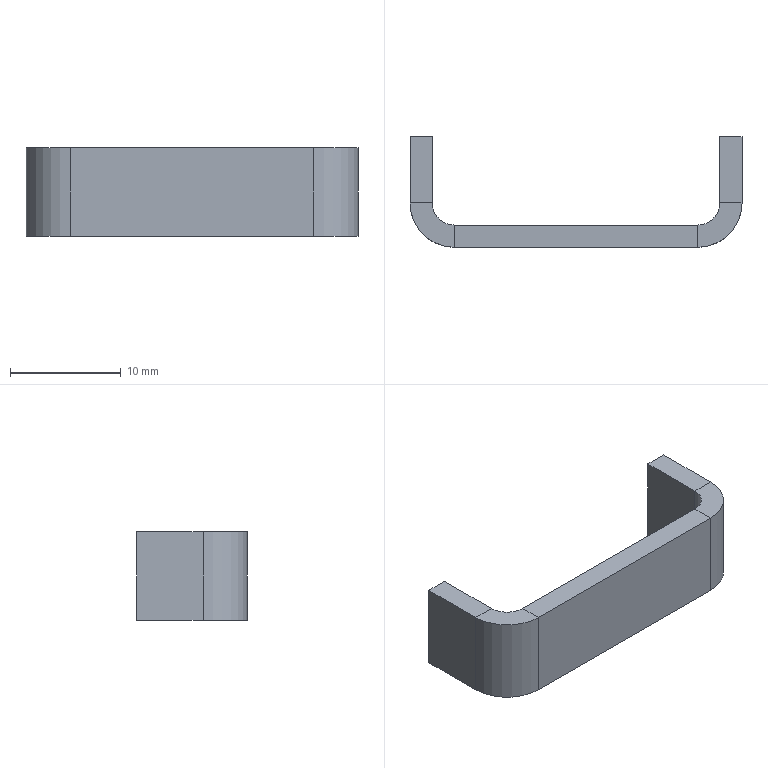Component | SolidWorks | ElectricalCabinetAssembly-1_ControlPanelAssembly-1_CableClamp-1 | 1 solid | 22 faces | box 30 x 10 x 8 mm | volume 695 mm3 | plane 18 | cylinder 4 | commonest cylinder face diameters 8 x2 4 x2 | material Plain Carbon Steel
STEP:
#1=COLOUR_RGB('',0.7922,0.8196,0.9333);
#2=FILL_AREA_STYLE_COLOUR('',#1);
#3=FILL_AREA_STYLE('',(#2));
#4=SURFACE_STYLE_FILL_AREA(#3);
#5=SURFACE_SIDE_STYLE('',(#4));
#6=SURFACE_STYLE_USAGE(.BOTH.,#5);
#7=PRESENTATION_STYLE_ASSIGNMENT((#6));
#8=CARTESIAN_POINT('',(86.921,47.384,67.696));
#9=VERTEX_POINT('',#8);
#10=CARTESIAN_POINT('',(86.921,47.463,67.696));
#11=VERTEX_POINT('',#10);
#12=CARTESIAN_POINT('',(86.921,47.384,67.696));
#13=DIRECTION('',(-0.,1.,0.));
#14=VECTOR('',#13,39.37);
#15=LINE('',#12,#14);
#16=EDGE_CURVE('',#9,#11,#15,.T.);
#17=ORIENTED_EDGE('',*,*,#16,.F.);
#18=CARTESIAN_POINT('',(86.763,47.541,67.696));
#19=VERTEX_POINT('',#18);
#20=CARTESIAN_POINT('',(86.921,47.541,67.696));
#21=DIRECTION('',(0.,-0.,1.));
#22=DIRECTION('',(1.,0.,0.));
#23=AXIS2_PLACEMENT_3D('',#20,#21,#22);
#24=CIRCLE('',#23,0.1575);
#25=EDGE_CURVE('',#19,#9,#24,.T.);
#26=ORIENTED_EDGE('',*,*,#25,.F.);
#27=CARTESIAN_POINT('',(86.842,47.541,67.696));
#28=VERTEX_POINT('',#27);
#29=CARTESIAN_POINT('',(86.842,47.541,67.696));
#30=DIRECTION('',(-1.,-0.,0.));
#31=VECTOR('',#30,39.37);
#32=LINE('',#29,#31);
#33=EDGE_CURVE('',#28,#19,#32,.T.);
#34=ORIENTED_EDGE('',*,*,#33,.F.);
#35=CARTESIAN_POINT('',(86.921,47.541,67.696));
#36=DIRECTION('',(0.,-0.,1.));
#37=DIRECTION('',(1.,0.,0.));
#38=AXIS2_PLACEMENT_3D('',#35,#36,#37);
#39=CIRCLE('',#38,0.07874);
#40=EDGE_CURVE('',#28,#11,#39,.T.);
#41=ORIENTED_EDGE('',*,*,#40,.T.);
#42=EDGE_LOOP('',(#17,#26,#34,#41));
#43=FACE_OUTER_BOUND('',#42,.T.);
#44=CARTESIAN_POINT('',(86.921,47.384,67.696));
#45=DIRECTION('',(-0.,0.,-1.));
#46=DIRECTION('',(1.,0.,-0.));
#47=AXIS2_PLACEMENT_3D('',#44,#45,#46);
#48=PLANE('',#47);
#49=ADVANCED_FACE('',(#43),#48,.T.);
#50=CARTESIAN_POINT('',(87.787,47.384,67.696));
#51=VERTEX_POINT('',#50);
#52=CARTESIAN_POINT('',(86.763,47.384,67.696));
#53=DIRECTION('',(1.,0.,-0.));
#54=VECTOR('',#53,39.37);
#55=LINE('',#52,#54);
#56=EDGE_CURVE('',#9,#51,#55,.T.);
#57=ORIENTED_EDGE('',*,*,#56,.F.);
#58=ORIENTED_EDGE('',*,*,#16,.T.);
#59=CARTESIAN_POINT('',(87.787,47.463,67.696));
#60=VERTEX_POINT('',#59);
#61=CARTESIAN_POINT('',(86.763,47.463,67.696));
#62=DIRECTION('',(1.,0.,-0.));
#63=VECTOR('',#62,39.37);
#64=LINE('',#61,#63);
#65=EDGE_CURVE('',#11,#60,#64,.T.);
#66=ORIENTED_EDGE('',*,*,#65,.T.);
#67=CARTESIAN_POINT('',(87.787,47.463,67.696));
#68=DIRECTION('',(0.,-1.,-0.));
#69=VECTOR('',#68,39.37);
#70=LINE('',#67,#69);
#71=EDGE_CURVE('',#60,#51,#70,.T.);
#72=ORIENTED_EDGE('',*,*,#71,.T.);
#73=EDGE_LOOP('',(#57,#58,#66,#72));
#74=FACE_OUTER_BOUND('',#73,.T.);
#75=CARTESIAN_POINT('',(86.842,47.541,67.696));
#76=DIRECTION('',(-0.,0.,-1.));
#77=DIRECTION('',(1.,0.,-0.));
#78=AXIS2_PLACEMENT_3D('',#75,#76,#77);
#79=PLANE('',#78);
#80=ADVANCED_FACE('',(#74),#79,.T.);
#81=CARTESIAN_POINT('',(86.763,47.541,68.011));
#82=VERTEX_POINT('',#81);
#83=CARTESIAN_POINT('',(86.842,47.541,68.011));
#84=VERTEX_POINT('',#83);
#85=CARTESIAN_POINT('',(86.763,47.541,68.011));
#86=DIRECTION('',(1.,0.,-0.));
#87=VECTOR('',#86,39.37);
#88=LINE('',#85,#87);
#89=EDGE_CURVE('',#82,#84,#88,.T.);
#90=ORIENTED_EDGE('',*,*,#89,.F.);
#91=CARTESIAN_POINT('',(86.921,47.384,68.011));
#92=VERTEX_POINT('',#91);
#93=CARTESIAN_POINT('',(86.921,47.541,68.011));
#94=DIRECTION('',(0.,-0.,1.));
#95=DIRECTION('',(1.,0.,0.));
#96=AXIS2_PLACEMENT_3D('',#93,#94,#95);
#97=CIRCLE('',#96,0.1575);
#98=EDGE_CURVE('',#82,#92,#97,.T.);
#99=ORIENTED_EDGE('',*,*,#98,.T.);
#100=CARTESIAN_POINT('',(86.921,47.463,68.011));
#101=VERTEX_POINT('',#100);
#102=CARTESIAN_POINT('',(86.921,47.463,68.011));
#103=DIRECTION('',(0.,-1.,-0.));
#104=VECTOR('',#103,39.37);
#105=LINE('',#102,#104);
#106=EDGE_CURVE('',#101,#92,#105,.T.);
#107=ORIENTED_EDGE('',*,*,#106,.F.);
#108=CARTESIAN_POINT('',(86.921,47.541,68.011));
#109=DIRECTION('',(0.,-0.,1.));
#110=DIRECTION('',(1.,0.,0.));
#111=AXIS2_PLACEMENT_3D('',#108,#109,#110);
#112=CIRCLE('',#111,0.07874);
#113=EDGE_CURVE('',#84,#101,#112,.T.);
#114=ORIENTED_EDGE('',*,*,#113,.F.);
#115=EDGE_LOOP('',(#90,#99,#107,#114));
#116=FACE_OUTER_BOUND('',#115,.T.);
#117=CARTESIAN_POINT('',(86.763,47.541,68.011));
#118=DIRECTION('',(0.,-0.,1.));
#119=DIRECTION('',(-1.,-0.,0.));
#120=AXIS2_PLACEMENT_3D('',#117,#118,#119);
#121=PLANE('',#120);
#122=ADVANCED_FACE('',(#116),#121,.T.);
#123=CARTESIAN_POINT('',(86.763,47.778,68.011));
#124=VERTEX_POINT('',#123);
#125=CARTESIAN_POINT('',(86.763,47.778,68.011));
#126=DIRECTION('',(0.,-1.,-0.));
#127=VECTOR('',#126,39.37);
#128=LINE('',#125,#127);
#129=EDGE_CURVE('',#124,#82,#128,.T.);
#130=ORIENTED_EDGE('',*,*,#129,.T.);
#131=ORIENTED_EDGE('',*,*,#89,.T.);
#132=CARTESIAN_POINT('',(86.842,47.778,68.011));
#133=VERTEX_POINT('',#132);
#134=CARTESIAN_POINT('',(86.842,47.778,68.011));
#135=DIRECTION('',(0.,-1.,-0.));
#136=VECTOR('',#135,39.37);
#137=LINE('',#134,#136);
#138=EDGE_CURVE('',#133,#84,#137,.T.);
#139=ORIENTED_EDGE('',*,*,#138,.F.);
#140=CARTESIAN_POINT('',(86.842,47.778,68.011));
#141=DIRECTION('',(-1.,-0.,0.));
#142=VECTOR('',#141,39.37);
#143=LINE('',#140,#142);
#144=EDGE_CURVE('',#133,#124,#143,.T.);
#145=ORIENTED_EDGE('',*,*,#144,.T.);
#146=EDGE_LOOP('',(#130,#131,#139,#145));
#147=FACE_OUTER_BOUND('',#146,.T.);
#148=CARTESIAN_POINT('',(86.921,47.463,68.011));
#149=DIRECTION('',(0.,-0.,1.));
#150=DIRECTION('',(-1.,-0.,0.));
#151=AXIS2_PLACEMENT_3D('',#148,#149,#150);
#152=PLANE('',#151);
#153=ADVANCED_FACE('',(#147),#152,.T.);
#154=CARTESIAN_POINT('',(87.944,47.541,67.696));
#155=VERTEX_POINT('',#154);
#156=CARTESIAN_POINT('',(87.866,47.541,67.696));
#157=VERTEX_POINT('',#156);
#158=CARTESIAN_POINT('',(87.944,47.541,67.696));
#159=DIRECTION('',(-1.,-0.,0.));
#160=VECTOR('',#159,39.37);
#161=LINE('',#158,#160);
#162=EDGE_CURVE('',#155,#157,#161,.T.);
#163=ORIENTED_EDGE('',*,*,#162,.F.);
#164=CARTESIAN_POINT('',(87.787,47.541,67.696));
#165=DIRECTION('',(0.,-0.,1.));
#166=DIRECTION('',(1.,0.,0.));
#167=AXIS2_PLACEMENT_3D('',#164,#165,#166);
#168=CIRCLE('',#167,0.1575);
#169=EDGE_CURVE('',#51,#155,#168,.T.);
#170=ORIENTED_EDGE('',*,*,#169,.F.);
#171=ORIENTED_EDGE('',*,*,#71,.F.);
#172=CARTESIAN_POINT('',(87.787,47.541,67.696));
#173=DIRECTION('',(0.,-0.,1.));
#174=DIRECTION('',(1.,0.,0.));
#175=AXIS2_PLACEMENT_3D('',#172,#173,#174);
#176=CIRCLE('',#175,0.07874);
#177=EDGE_CURVE('',#60,#157,#176,.T.);
#178=ORIENTED_EDGE('',*,*,#177,.T.);
#179=EDGE_LOOP('',(#163,#170,#171,#178));
#180=FACE_OUTER_BOUND('',#179,.T.);
#181=CARTESIAN_POINT('',(87.944,47.541,67.696));
#182=DIRECTION('',(-0.,0.,-1.));
#183=DIRECTION('',(1.,0.,-0.));
#184=AXIS2_PLACEMENT_3D('',#181,#182,#183);
#185=PLANE('',#184);
#186=ADVANCED_FACE('',(#180),#185,.T.);
#187=CARTESIAN_POINT('',(87.944,47.778,67.696));
#188=VERTEX_POINT('',#187);
#189=CARTESIAN_POINT('',(87.944,47.384,67.696));
#190=DIRECTION('',(-0.,1.,0.));
#191=VECTOR('',#190,39.37);
#192=LINE('',#189,#191);
#193=EDGE_CURVE('',#155,#188,#192,.T.);
#194=ORIENTED_EDGE('',*,*,#193,.F.);
#195=ORIENTED_EDGE('',*,*,#162,.T.);
#196=CARTESIAN_POINT('',(87.866,47.778,67.696));
#197=VERTEX_POINT('',#196);
#198=CARTESIAN_POINT('',(87.866,47.384,67.696));
#199=DIRECTION('',(-0.,1.,0.));
#200=VECTOR('',#199,39.37);
#201=LINE('',#198,#200);
#202=EDGE_CURVE('',#157,#197,#201,.T.);
#203=ORIENTED_EDGE('',*,*,#202,.T.);
#204=CARTESIAN_POINT('',(87.944,47.778,67.696));
#205=DIRECTION('',(-1.,-0.,0.));
#206=VECTOR('',#205,39.37);
#207=LINE('',#204,#206);
#208=EDGE_CURVE('',#188,#197,#207,.T.);
#209=ORIENTED_EDGE('',*,*,#208,.F.);
#210=EDGE_LOOP('',(#194,#195,#203,#209));
#211=FACE_OUTER_BOUND('',#210,.T.);
#212=CARTESIAN_POINT('',(87.787,47.463,67.696));
#213=DIRECTION('',(-0.,0.,-1.));
#214=DIRECTION('',(1.,0.,-0.));
#215=AXIS2_PLACEMENT_3D('',#212,#213,#214);
#216=PLANE('',#215);
#217=ADVANCED_FACE('',(#211),#216,.T.);
#218=CARTESIAN_POINT('',(87.787,47.384,68.011));
#219=VERTEX_POINT('',#218);
#220=CARTESIAN_POINT('',(87.787,47.463,68.011));
#221=VERTEX_POINT('',#220);
#222=CARTESIAN_POINT('',(87.787,47.384,68.011));
#223=DIRECTION('',(-0.,1.,0.));
#224=VECTOR('',#223,39.37);
#225=LINE('',#222,#224);
#226=EDGE_CURVE('',#219,#221,#225,.T.);
#227=ORIENTED_EDGE('',*,*,#226,.F.);
#228=CARTESIAN_POINT('',(87.944,47.541,68.011));
#229=VERTEX_POINT('',#228);
#230=CARTESIAN_POINT('',(87.787,47.541,68.011));
#231=DIRECTION('',(0.,-0.,1.));
#232=DIRECTION('',(1.,0.,0.));
#233=AXIS2_PLACEMENT_3D('',#230,#231,#232);
#234=CIRCLE('',#233,0.1575);
#235=EDGE_CURVE('',#219,#229,#234,.T.);
#236=ORIENTED_EDGE('',*,*,#235,.T.);
#237=CARTESIAN_POINT('',(87.866,47.541,68.011));
#238=VERTEX_POINT('',#237);
#239=CARTESIAN_POINT('',(87.866,47.541,68.011));
#240=DIRECTION('',(1.,0.,-0.));
#241=VECTOR('',#240,39.37);
#242=LINE('',#239,#241);
#243=EDGE_CURVE('',#238,#229,#242,.T.);
#244=ORIENTED_EDGE('',*,*,#243,.F.);
#245=CARTESIAN_POINT('',(87.787,47.541,68.011));
#246=DIRECTION('',(0.,-0.,1.));
#247=DIRECTION('',(1.,0.,0.));
#248=AXIS2_PLACEMENT_3D('',#245,#246,#247);
#249=CIRCLE('',#248,0.07874);
#250=EDGE_CURVE('',#221,#238,#249,.T.);
#251=ORIENTED_EDGE('',*,*,#250,.F.);
#252=EDGE_LOOP('',(#227,#236,#244,#251));
#253=FACE_OUTER_BOUND('',#252,.T.);
#254=CARTESIAN_POINT('',(87.787,47.384,68.011));
#255=DIRECTION('',(0.,-0.,1.));
#256=DIRECTION('',(-1.,-0.,0.));
#257=AXIS2_PLACEMENT_3D('',#254,#255,#256);
#258=PLANE('',#257);
#259=ADVANCED_FACE('',(#253),#258,.T.);
#260=CARTESIAN_POINT('',(86.763,47.384,68.011));
#261=DIRECTION('',(1.,0.,-0.));
#262=VECTOR('',#261,39.37);
#263=LINE('',#260,#262);
#264=EDGE_CURVE('',#92,#219,#263,.T.);
#265=ORIENTED_EDGE('',*,*,#264,.T.);
#266=ORIENTED_EDGE('',*,*,#226,.T.);
#267=CARTESIAN_POINT('',(86.763,47.463,68.011));
#268=DIRECTION('',(1.,0.,-0.));
#269=VECTOR('',#268,39.37);
#270=LINE('',#267,#269);
#271=EDGE_CURVE('',#101,#221,#270,.T.);
#272=ORIENTED_EDGE('',*,*,#271,.F.);
#273=ORIENTED_EDGE('',*,*,#106,.T.);
#274=EDGE_LOOP('',(#265,#266,#272,#273));
#275=FACE_OUTER_BOUND('',#274,.T.);
#276=CARTESIAN_POINT('',(87.866,47.541,68.011));
#277=DIRECTION('',(0.,-0.,1.));
#278=DIRECTION('',(-1.,-0.,0.));
#279=AXIS2_PLACEMENT_3D('',#276,#277,#278);
#280=PLANE('',#279);
#281=ADVANCED_FACE('',(#275),#280,.T.);
#282=CARTESIAN_POINT('',(87.866,47.778,68.011));
#283=VERTEX_POINT('',#282);
#284=CARTESIAN_POINT('',(87.866,47.384,68.011));
#285=DIRECTION('',(-0.,1.,0.));
#286=VECTOR('',#285,39.37);
#287=LINE('',#284,#286);
#288=EDGE_CURVE('',#238,#283,#287,.T.);
#289=ORIENTED_EDGE('',*,*,#288,.T.);
#290=CARTESIAN_POINT('',(87.866,47.778,67.696));
#291=DIRECTION('',(0.,-0.,1.));
#292=VECTOR('',#291,39.37);
#293=LINE('',#290,#292);
#294=EDGE_CURVE('',#197,#283,#293,.T.);
#295=ORIENTED_EDGE('',*,*,#294,.F.);
#296=ORIENTED_EDGE('',*,*,#202,.F.);
#297=CARTESIAN_POINT('',(87.866,47.541,67.696));
#298=DIRECTION('',(0.,-0.,1.));
#299=VECTOR('',#298,39.37);
#300=LINE('',#297,#299);
#301=EDGE_CURVE('',#157,#238,#300,.T.);
#302=ORIENTED_EDGE('',*,*,#301,.T.);
#303=EDGE_LOOP('',(#289,#295,#296,#302));
#304=FACE_OUTER_BOUND('',#303,.T.);
#305=CARTESIAN_POINT('',(87.866,47.384,67.696));
#306=DIRECTION('',(1.,0.,-0.));
#307=DIRECTION('',(0.,-1.,-0.));
#308=AXIS2_PLACEMENT_3D('',#305,#306,#307);
#309=PLANE('',#308);
#310=ADVANCED_FACE('',(#304),#309,.F.);
#311=CARTESIAN_POINT('',(87.944,47.778,68.011));
#312=VERTEX_POINT('',#311);
#313=CARTESIAN_POINT('',(87.944,47.778,68.011));
#314=DIRECTION('',(-1.,-0.,0.));
#315=VECTOR('',#314,39.37);
#316=LINE('',#313,#315);
#317=EDGE_CURVE('',#312,#283,#316,.T.);
#318=ORIENTED_EDGE('',*,*,#317,.F.);
#319=CARTESIAN_POINT('',(87.944,47.778,67.696));
#320=DIRECTION('',(0.,-0.,1.));
#321=VECTOR('',#320,39.37);
#322=LINE('',#319,#321);
#323=EDGE_CURVE('',#188,#312,#322,.T.);
#324=ORIENTED_EDGE('',*,*,#323,.F.);
#325=ORIENTED_EDGE('',*,*,#208,.T.);
#326=ORIENTED_EDGE('',*,*,#294,.T.);
#327=EDGE_LOOP('',(#318,#324,#325,#326));
#328=FACE_OUTER_BOUND('',#327,.T.);
#329=CARTESIAN_POINT('',(87.944,47.778,67.696));
#330=DIRECTION('',(-0.,1.,0.));
#331=DIRECTION('',(0.,-0.,1.));
#332=AXIS2_PLACEMENT_3D('',#329,#330,#331);
#333=PLANE('',#332);
#334=ADVANCED_FACE('',(#328),#333,.T.);
#335=CARTESIAN_POINT('',(87.944,47.384,68.011));
#336=DIRECTION('',(-0.,1.,0.));
#337=VECTOR('',#336,39.37);
#338=LINE('',#335,#337);
#339=EDGE_CURVE('',#229,#312,#338,.T.);
#340=ORIENTED_EDGE('',*,*,#339,.F.);
#341=CARTESIAN_POINT('',(87.944,47.541,67.696));
#342=DIRECTION('',(0.,-0.,1.));
#343=VECTOR('',#342,39.37);
#344=LINE('',#341,#343);
#345=EDGE_CURVE('',#155,#229,#344,.T.);
#346=ORIENTED_EDGE('',*,*,#345,.F.);
#347=ORIENTED_EDGE('',*,*,#193,.T.);
#348=ORIENTED_EDGE('',*,*,#323,.T.);
#349=EDGE_LOOP('',(#340,#346,#347,#348));
#350=FACE_OUTER_BOUND('',#349,.T.);
#351=CARTESIAN_POINT('',(87.944,47.384,67.696));
#352=DIRECTION('',(1.,0.,-0.));
#353=DIRECTION('',(0.,-1.,-0.));
#354=AXIS2_PLACEMENT_3D('',#351,#352,#353);
#355=PLANE('',#354);
#356=ADVANCED_FACE('',(#350),#355,.T.);
#357=ORIENTED_EDGE('',*,*,#235,.F.);
#358=CARTESIAN_POINT('',(87.787,47.384,67.696));
#359=DIRECTION('',(0.,-0.,1.));
#360=VECTOR('',#359,39.37);
#361=LINE('',#358,#360);
#362=EDGE_CURVE('',#51,#219,#361,.T.);
#363=ORIENTED_EDGE('',*,*,#362,.F.);
#364=ORIENTED_EDGE('',*,*,#169,.T.);
#365=ORIENTED_EDGE('',*,*,#345,.T.);
#366=EDGE_LOOP('',(#357,#363,#364,#365));
#367=FACE_OUTER_BOUND('',#366,.T.);
#368=CARTESIAN_POINT('',(87.787,47.541,67.696));
#369=DIRECTION('',(0.,-0.,1.));
#370=DIRECTION('',(-1.,0.,0.));
#371=AXIS2_PLACEMENT_3D('',#368,#369,#370);
#372=CYLINDRICAL_SURFACE('',#371,0.1575);
#373=ADVANCED_FACE('',(#367),#372,.T.);
#374=ORIENTED_EDGE('',*,*,#264,.F.);
#375=CARTESIAN_POINT('',(86.921,47.384,67.696));
#376=DIRECTION('',(0.,-0.,1.));
#377=VECTOR('',#376,39.37);
#378=LINE('',#375,#377);
#379=EDGE_CURVE('',#9,#92,#378,.T.);
#380=ORIENTED_EDGE('',*,*,#379,.F.);
#381=ORIENTED_EDGE('',*,*,#56,.T.);
#382=ORIENTED_EDGE('',*,*,#362,.T.);
#383=EDGE_LOOP('',(#374,#380,#381,#382));
#384=FACE_OUTER_BOUND('',#383,.T.);
#385=CARTESIAN_POINT('',(86.763,47.384,67.696));
#386=DIRECTION('',(0.,-1.,-0.));
#387=DIRECTION('',(-0.,0.,-1.));
#388=AXIS2_PLACEMENT_3D('',#385,#386,#387);
#389=PLANE('',#388);
#390=ADVANCED_FACE('',(#384),#389,.T.);
#391=ORIENTED_EDGE('',*,*,#98,.F.);
#392=CARTESIAN_POINT('',(86.763,47.541,67.696));
#393=DIRECTION('',(0.,-0.,1.));
#394=VECTOR('',#393,39.37);
#395=LINE('',#392,#394);
#396=EDGE_CURVE('',#19,#82,#395,.T.);
#397=ORIENTED_EDGE('',*,*,#396,.F.);
#398=ORIENTED_EDGE('',*,*,#25,.T.);
#399=ORIENTED_EDGE('',*,*,#379,.T.);
#400=EDGE_LOOP('',(#391,#397,#398,#399));
#401=FACE_OUTER_BOUND('',#400,.T.);
#402=CARTESIAN_POINT('',(86.921,47.541,67.696));
#403=DIRECTION('',(0.,-0.,1.));
#404=DIRECTION('',(-1.,0.,0.));
#405=AXIS2_PLACEMENT_3D('',#402,#403,#404);
#406=CYLINDRICAL_SURFACE('',#405,0.1575);
#407=ADVANCED_FACE('',(#401),#406,.T.);
#408=ORIENTED_EDGE('',*,*,#129,.F.);
#409=CARTESIAN_POINT('',(86.763,47.778,67.696));
#410=VERTEX_POINT('',#409);
#411=CARTESIAN_POINT('',(86.763,47.778,67.696));
#412=DIRECTION('',(0.,-0.,1.));
#413=VECTOR('',#412,39.37);
#414=LINE('',#411,#413);
#415=EDGE_CURVE('',#410,#124,#414,.T.);
#416=ORIENTED_EDGE('',*,*,#415,.F.);
#417=CARTESIAN_POINT('',(86.763,47.778,67.696));
#418=DIRECTION('',(0.,-1.,-0.));
#419=VECTOR('',#418,39.37);
#420=LINE('',#417,#419);
#421=EDGE_CURVE('',#410,#19,#420,.T.);
#422=ORIENTED_EDGE('',*,*,#421,.T.);
#423=ORIENTED_EDGE('',*,*,#396,.T.);
#424=EDGE_LOOP('',(#408,#416,#422,#423));
#425=FACE_OUTER_BOUND('',#424,.T.);
#426=CARTESIAN_POINT('',(86.763,47.778,67.696));
#427=DIRECTION('',(-1.,-0.,0.));
#428=DIRECTION('',(-0.,0.,-1.));
#429=AXIS2_PLACEMENT_3D('',#426,#427,#428);
#430=PLANE('',#429);
#431=ADVANCED_FACE('',(#425),#430,.T.);
#432=ORIENTED_EDGE('',*,*,#144,.F.);
#433=CARTESIAN_POINT('',(86.842,47.778,67.696));
#434=VERTEX_POINT('',#433);
#435=CARTESIAN_POINT('',(86.842,47.778,67.696));
#436=DIRECTION('',(0.,-0.,1.));
#437=VECTOR('',#436,39.37);
#438=LINE('',#435,#437);
#439=EDGE_CURVE('',#434,#133,#438,.T.);
#440=ORIENTED_EDGE('',*,*,#439,.F.);
#441=CARTESIAN_POINT('',(86.842,47.778,67.696));
#442=DIRECTION('',(-1.,-0.,0.));
#443=VECTOR('',#442,39.37);
#444=LINE('',#441,#443);
#445=EDGE_CURVE('',#434,#410,#444,.T.);
#446=ORIENTED_EDGE('',*,*,#445,.T.);
#447=ORIENTED_EDGE('',*,*,#415,.T.);
#448=EDGE_LOOP('',(#432,#440,#446,#447));
#449=FACE_OUTER_BOUND('',#448,.T.);
#450=CARTESIAN_POINT('',(86.842,47.778,67.696));
#451=DIRECTION('',(-0.,1.,0.));
#452=DIRECTION('',(0.,-0.,1.));
#453=AXIS2_PLACEMENT_3D('',#450,#451,#452);
#454=PLANE('',#453);
#455=ADVANCED_FACE('',(#449),#454,.T.);
#456=ORIENTED_EDGE('',*,*,#138,.T.);
#457=CARTESIAN_POINT('',(86.842,47.541,67.696));
#458=DIRECTION('',(0.,-0.,1.));
#459=VECTOR('',#458,39.37);
#460=LINE('',#457,#459);
#461=EDGE_CURVE('',#28,#84,#460,.T.);
#462=ORIENTED_EDGE('',*,*,#461,.F.);
#463=CARTESIAN_POINT('',(86.842,47.778,67.696));
#464=DIRECTION('',(0.,-1.,-0.));
#465=VECTOR('',#464,39.37);
#466=LINE('',#463,#465);
#467=EDGE_CURVE('',#434,#28,#466,.T.);
#468=ORIENTED_EDGE('',*,*,#467,.F.);
#469=ORIENTED_EDGE('',*,*,#439,.T.);
#470=EDGE_LOOP('',(#456,#462,#468,#469));
#471=FACE_OUTER_BOUND('',#470,.T.);
#472=CARTESIAN_POINT('',(86.842,47.778,67.696));
#473=DIRECTION('',(-1.,-0.,0.));
#474=DIRECTION('',(-0.,0.,-1.));
#475=AXIS2_PLACEMENT_3D('',#472,#473,#474);
#476=PLANE('',#475);
#477=ADVANCED_FACE('',(#471),#476,.F.);
#478=ORIENTED_EDGE('',*,*,#113,.T.);
#479=CARTESIAN_POINT('',(86.921,47.463,67.696));
#480=DIRECTION('',(0.,-0.,1.));
#481=VECTOR('',#480,39.37);
#482=LINE('',#479,#481);
#483=EDGE_CURVE('',#11,#101,#482,.T.);
#484=ORIENTED_EDGE('',*,*,#483,.F.);
#485=ORIENTED_EDGE('',*,*,#40,.F.);
#486=ORIENTED_EDGE('',*,*,#461,.T.);
#487=EDGE_LOOP('',(#478,#484,#485,#486));
#488=FACE_OUTER_BOUND('',#487,.T.);
#489=CARTESIAN_POINT('',(86.921,47.541,67.696));
#490=DIRECTION('',(0.,-0.,1.));
#491=DIRECTION('',(-1.,0.,0.));
#492=AXIS2_PLACEMENT_3D('',#489,#490,#491);
#493=CYLINDRICAL_SURFACE('',#492,0.07874);
#494=ADVANCED_FACE('',(#488),#493,.F.);
#495=ORIENTED_EDGE('',*,*,#271,.T.);
#496=CARTESIAN_POINT('',(87.787,47.463,67.696));
#497=DIRECTION('',(0.,-0.,1.));
#498=VECTOR('',#497,39.37);
#499=LINE('',#496,#498);
#500=EDGE_CURVE('',#60,#221,#499,.T.);
#501=ORIENTED_EDGE('',*,*,#500,.F.);
#502=ORIENTED_EDGE('',*,*,#65,.F.);
#503=ORIENTED_EDGE('',*,*,#483,.T.);
#504=EDGE_LOOP('',(#495,#501,#502,#503));
#505=FACE_OUTER_BOUND('',#504,.T.);
#506=CARTESIAN_POINT('',(86.763,47.463,67.696));
#507=DIRECTION('',(0.,-1.,-0.));
#508=DIRECTION('',(-0.,0.,-1.));
#509=AXIS2_PLACEMENT_3D('',#506,#507,#508);
#510=PLANE('',#509);
#511=ADVANCED_FACE('',(#505),#510,.F.);
#512=ORIENTED_EDGE('',*,*,#250,.T.);
#513=ORIENTED_EDGE('',*,*,#301,.F.);
#514=ORIENTED_EDGE('',*,*,#177,.F.);
#515=ORIENTED_EDGE('',*,*,#500,.T.);
#516=EDGE_LOOP('',(#512,#513,#514,#515));
#517=FACE_OUTER_BOUND('',#516,.T.);
#518=CARTESIAN_POINT('',(87.787,47.541,67.696));
#519=DIRECTION('',(0.,-0.,1.));
#520=DIRECTION('',(-1.,0.,0.));
#521=AXIS2_PLACEMENT_3D('',#518,#519,#520);
#522=CYLINDRICAL_SURFACE('',#521,0.07874);
#523=ADVANCED_FACE('',(#517),#522,.F.);
#524=ORIENTED_EDGE('',*,*,#467,.T.);
#525=ORIENTED_EDGE('',*,*,#33,.T.);
#526=ORIENTED_EDGE('',*,*,#421,.F.);
#527=ORIENTED_EDGE('',*,*,#445,.F.);
#528=EDGE_LOOP('',(#524,#525,#526,#527));
#529=FACE_OUTER_BOUND('',#528,.T.);
#530=CARTESIAN_POINT('',(87.787,47.541,67.696));
#531=DIRECTION('',(-0.,0.,-1.));
#532=DIRECTION('',(1.,0.,-0.));
#533=AXIS2_PLACEMENT_3D('',#530,#531,#532);
#534=PLANE('',#533);
#535=ADVANCED_FACE('',(#529),#534,.T.);
#536=ORIENTED_EDGE('',*,*,#288,.F.);
#537=ORIENTED_EDGE('',*,*,#243,.T.);
#538=ORIENTED_EDGE('',*,*,#339,.T.);
#539=ORIENTED_EDGE('',*,*,#317,.T.);
#540=EDGE_LOOP('',(#536,#537,#538,#539));
#541=FACE_OUTER_BOUND('',#540,.T.);
#542=CARTESIAN_POINT('',(87.787,47.541,68.011));
#543=DIRECTION('',(-0.,0.,-1.));
#544=DIRECTION('',(1.,0.,-0.));
#545=AXIS2_PLACEMENT_3D('',#542,#543,#544);
#546=PLANE('',#545);
#547=ADVANCED_FACE('',(#541),#546,.F.);
#548=CLOSED_SHELL('',(#49,#80,#122,#153,#186,#217,#259,#281,#310,#334,#356,#373,#390,#407,#431,#455,#477,#494,#511,#523,#535,#547));
#549=MANIFOLD_SOLID_BREP('',#548);
#550=STYLED_ITEM('',(#7),#549);
#551=(LENGTH_UNIT()NAMED_UNIT(*)SI_UNIT($,.METRE.));
#552=LENGTH_MEASURE_WITH_UNIT(LENGTH_MEASURE(0.0254),#551);
#553=DIMENSIONAL_EXPONENTS(1.,0.,0.,0.,0.,0.,0.);
#554=(CONVERSION_BASED_UNIT('',#552)LENGTH_UNIT()NAMED_UNIT(#553));
#555=UNCERTAINTY_MEASURE_WITH_UNIT(LENGTH_MEASURE(0.00001),#554,'','');
#556=(NAMED_UNIT(*)PLANE_ANGLE_UNIT()SI_UNIT($,.RADIAN.));
#557=(NAMED_UNIT(*)SI_UNIT($,.STERADIAN.)SOLID_ANGLE_UNIT());
#558=(GEOMETRIC_REPRESENTATION_CONTEXT(3)GLOBAL_UNCERTAINTY_ASSIGNED_CONTEXT((#555))GLOBAL_UNIT_ASSIGNED_CONTEXT((#554,#556,#557))REPRESENTATION_CONTEXT('',''));
#559=MECHANICAL_DESIGN_GEOMETRIC_PRESENTATION_REPRESENTATION('',(#550),#558);
#560=PRESENTATION_LAYER_ASSIGNMENT('','',(#550));
#561=CARTESIAN_POINT('',(0.,0.,0.));
#562=DIRECTION('',(0.,0.,1.));
#563=DIRECTION('',(1.,0.,0.));
#564=AXIS2_PLACEMENT_3D('',#561,#562,#563);
#565=(LENGTH_UNIT()NAMED_UNIT(*)SI_UNIT($,.METRE.));
#566=LENGTH_MEASURE_WITH_UNIT(LENGTH_MEASURE(0.0254),#565);
#567=DIMENSIONAL_EXPONENTS(1.,0.,0.,0.,0.,0.,0.);
#568=(CONVERSION_BASED_UNIT('',#566)LENGTH_UNIT()NAMED_UNIT(#567));
#569=UNCERTAINTY_MEASURE_WITH_UNIT(LENGTH_MEASURE(0.00001),#568,'','');
#570=(NAMED_UNIT(*)PLANE_ANGLE_UNIT()SI_UNIT($,.RADIAN.));
#571=(NAMED_UNIT(*)SI_UNIT($,.STERADIAN.)SOLID_ANGLE_UNIT());
#572=(GEOMETRIC_REPRESENTATION_CONTEXT(3)GLOBAL_UNCERTAINTY_ASSIGNED_CONTEXT((#569))GLOBAL_UNIT_ASSIGNED_CONTEXT((#568,#570,#571))REPRESENTATION_CONTEXT('',''));
#573=ADVANCED_BREP_SHAPE_REPRESENTATION('',(#549,#564),#572);